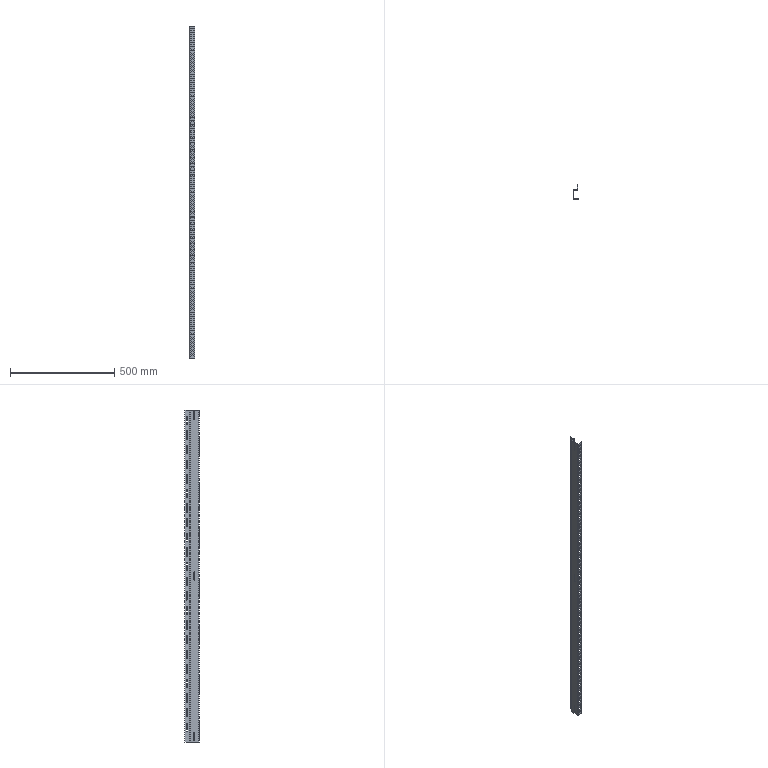Component | SolidWorks | InnerColumn-1 | 1 solid | 471 faces | volume 315901 mm3 | plane 390 | cylinder 81 | commonest cylinder face diameters 5 x75 2 x3 6 x3